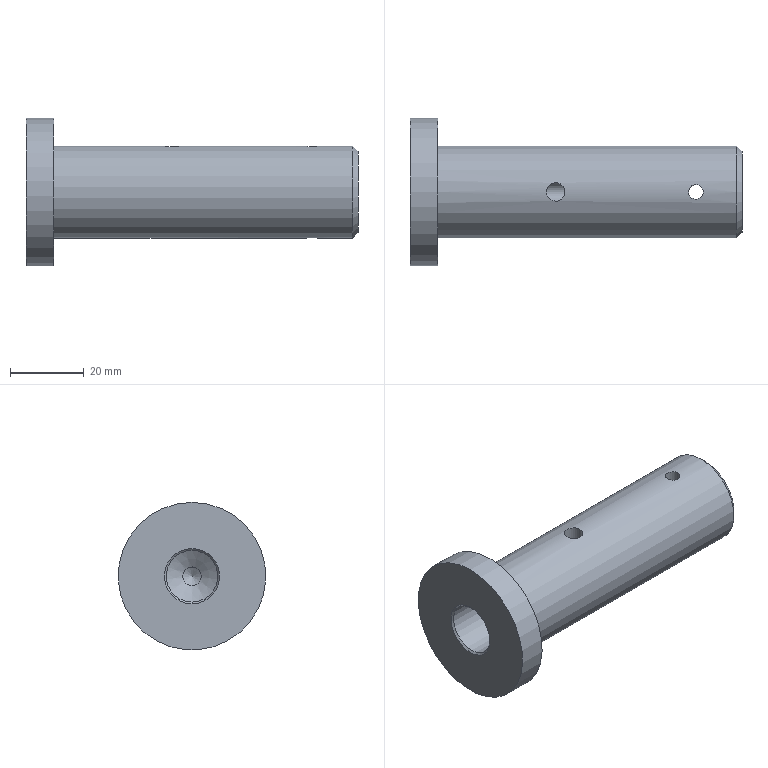Component | NX | 2_MANDREL | 1 solid | 13 faces | volume 44993 mm3 | cylinder 6 | cone 4 | plane 3 | commonest cylinder face diameters 5 x2 25 x1 40 x1 4 x1 14 x1